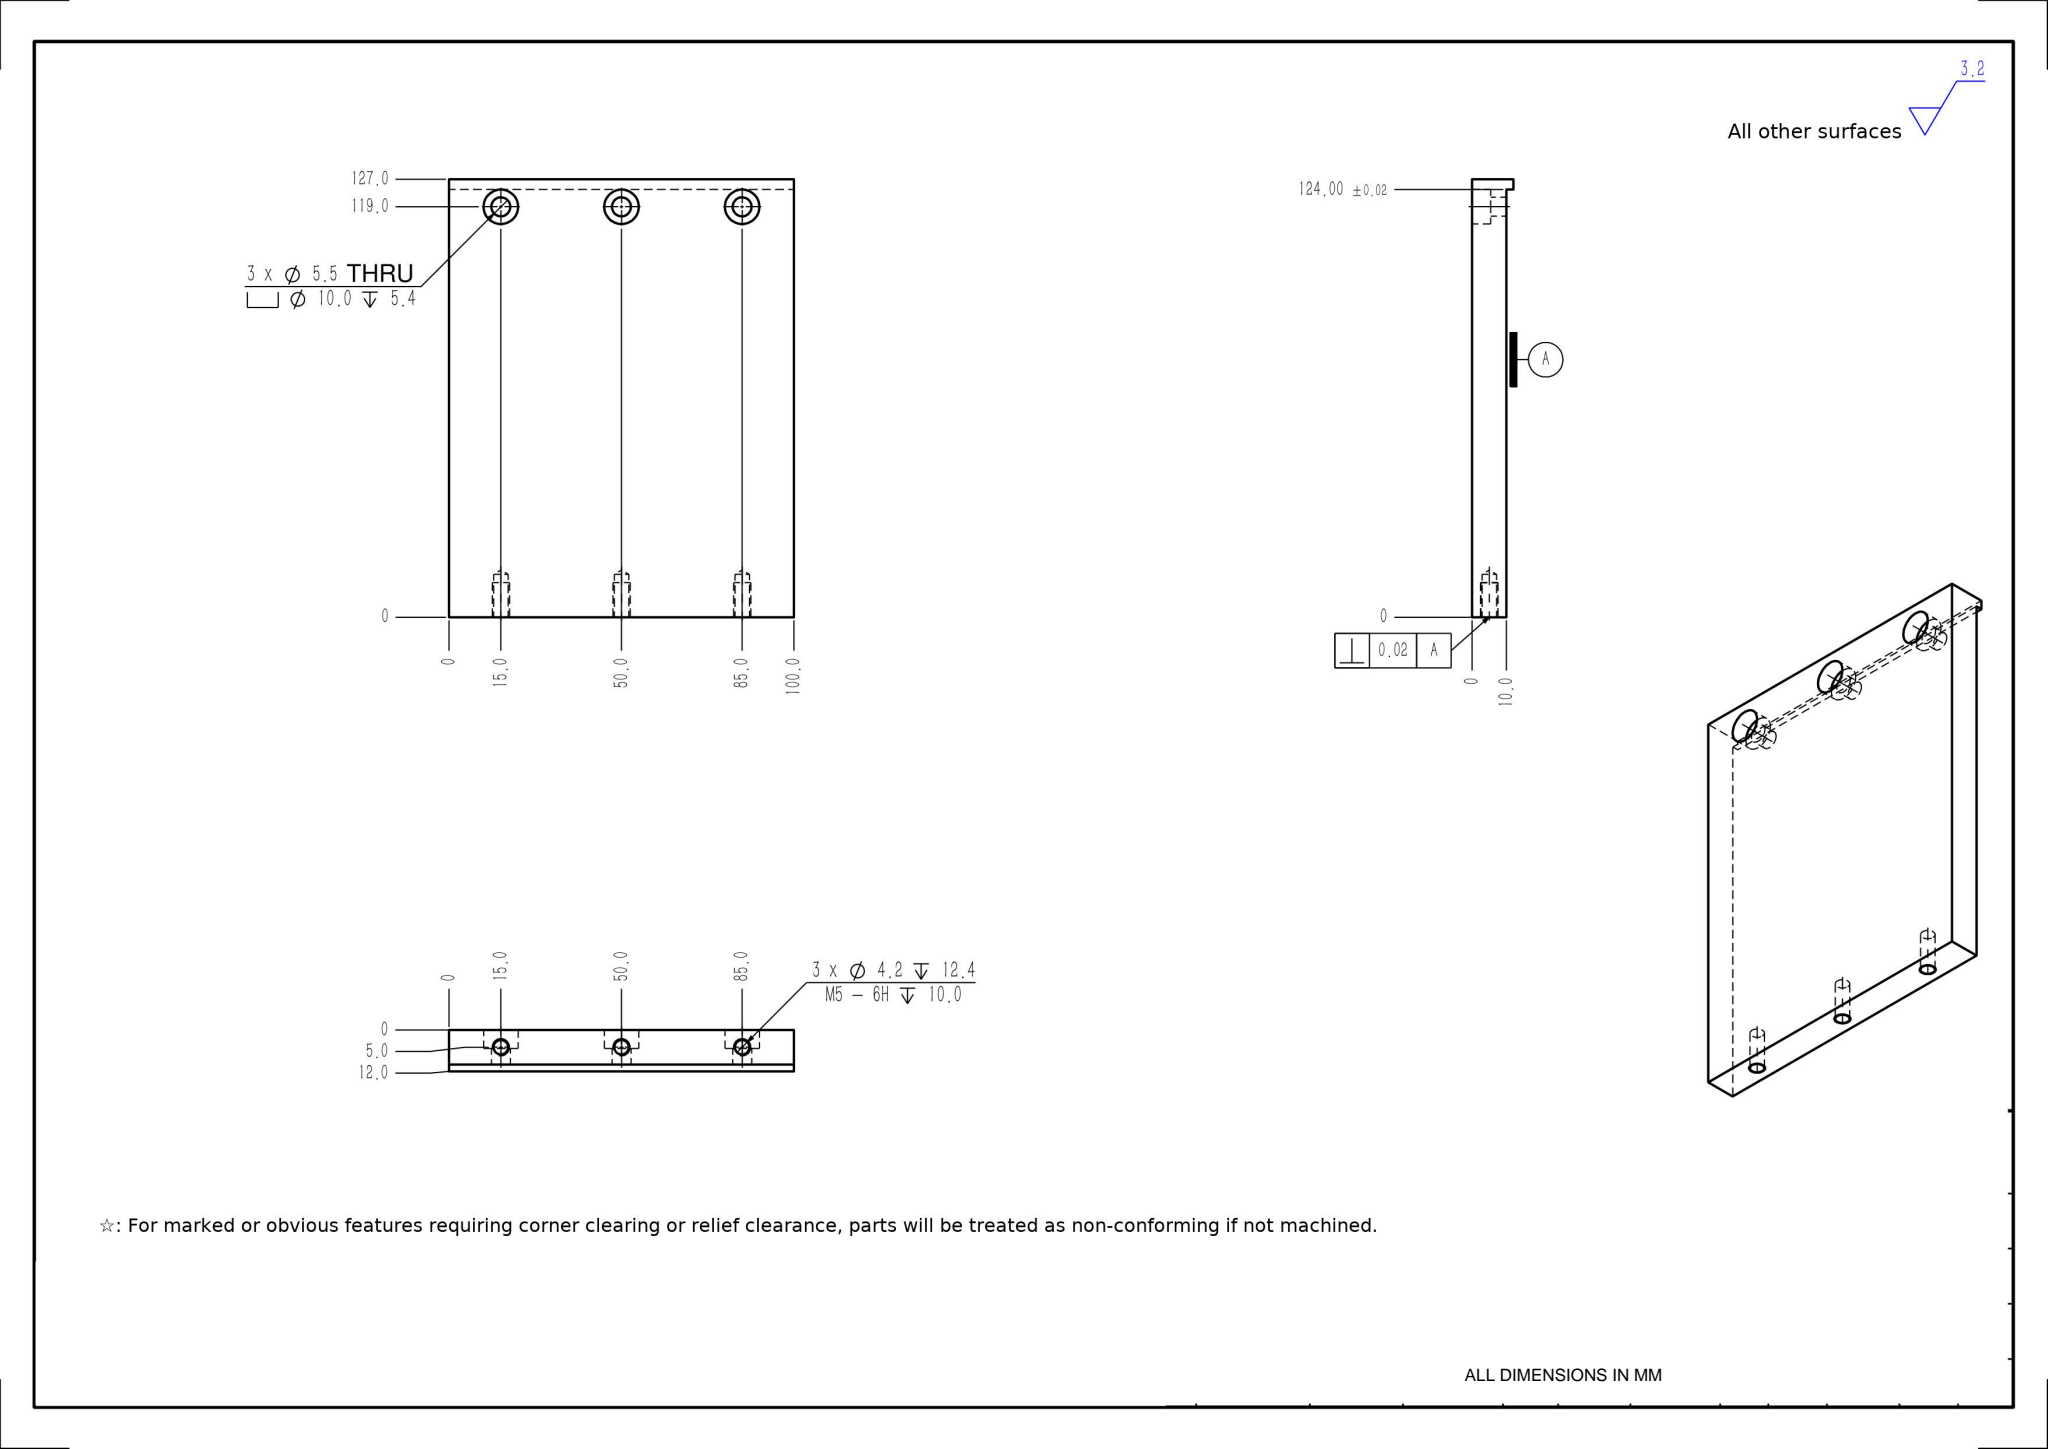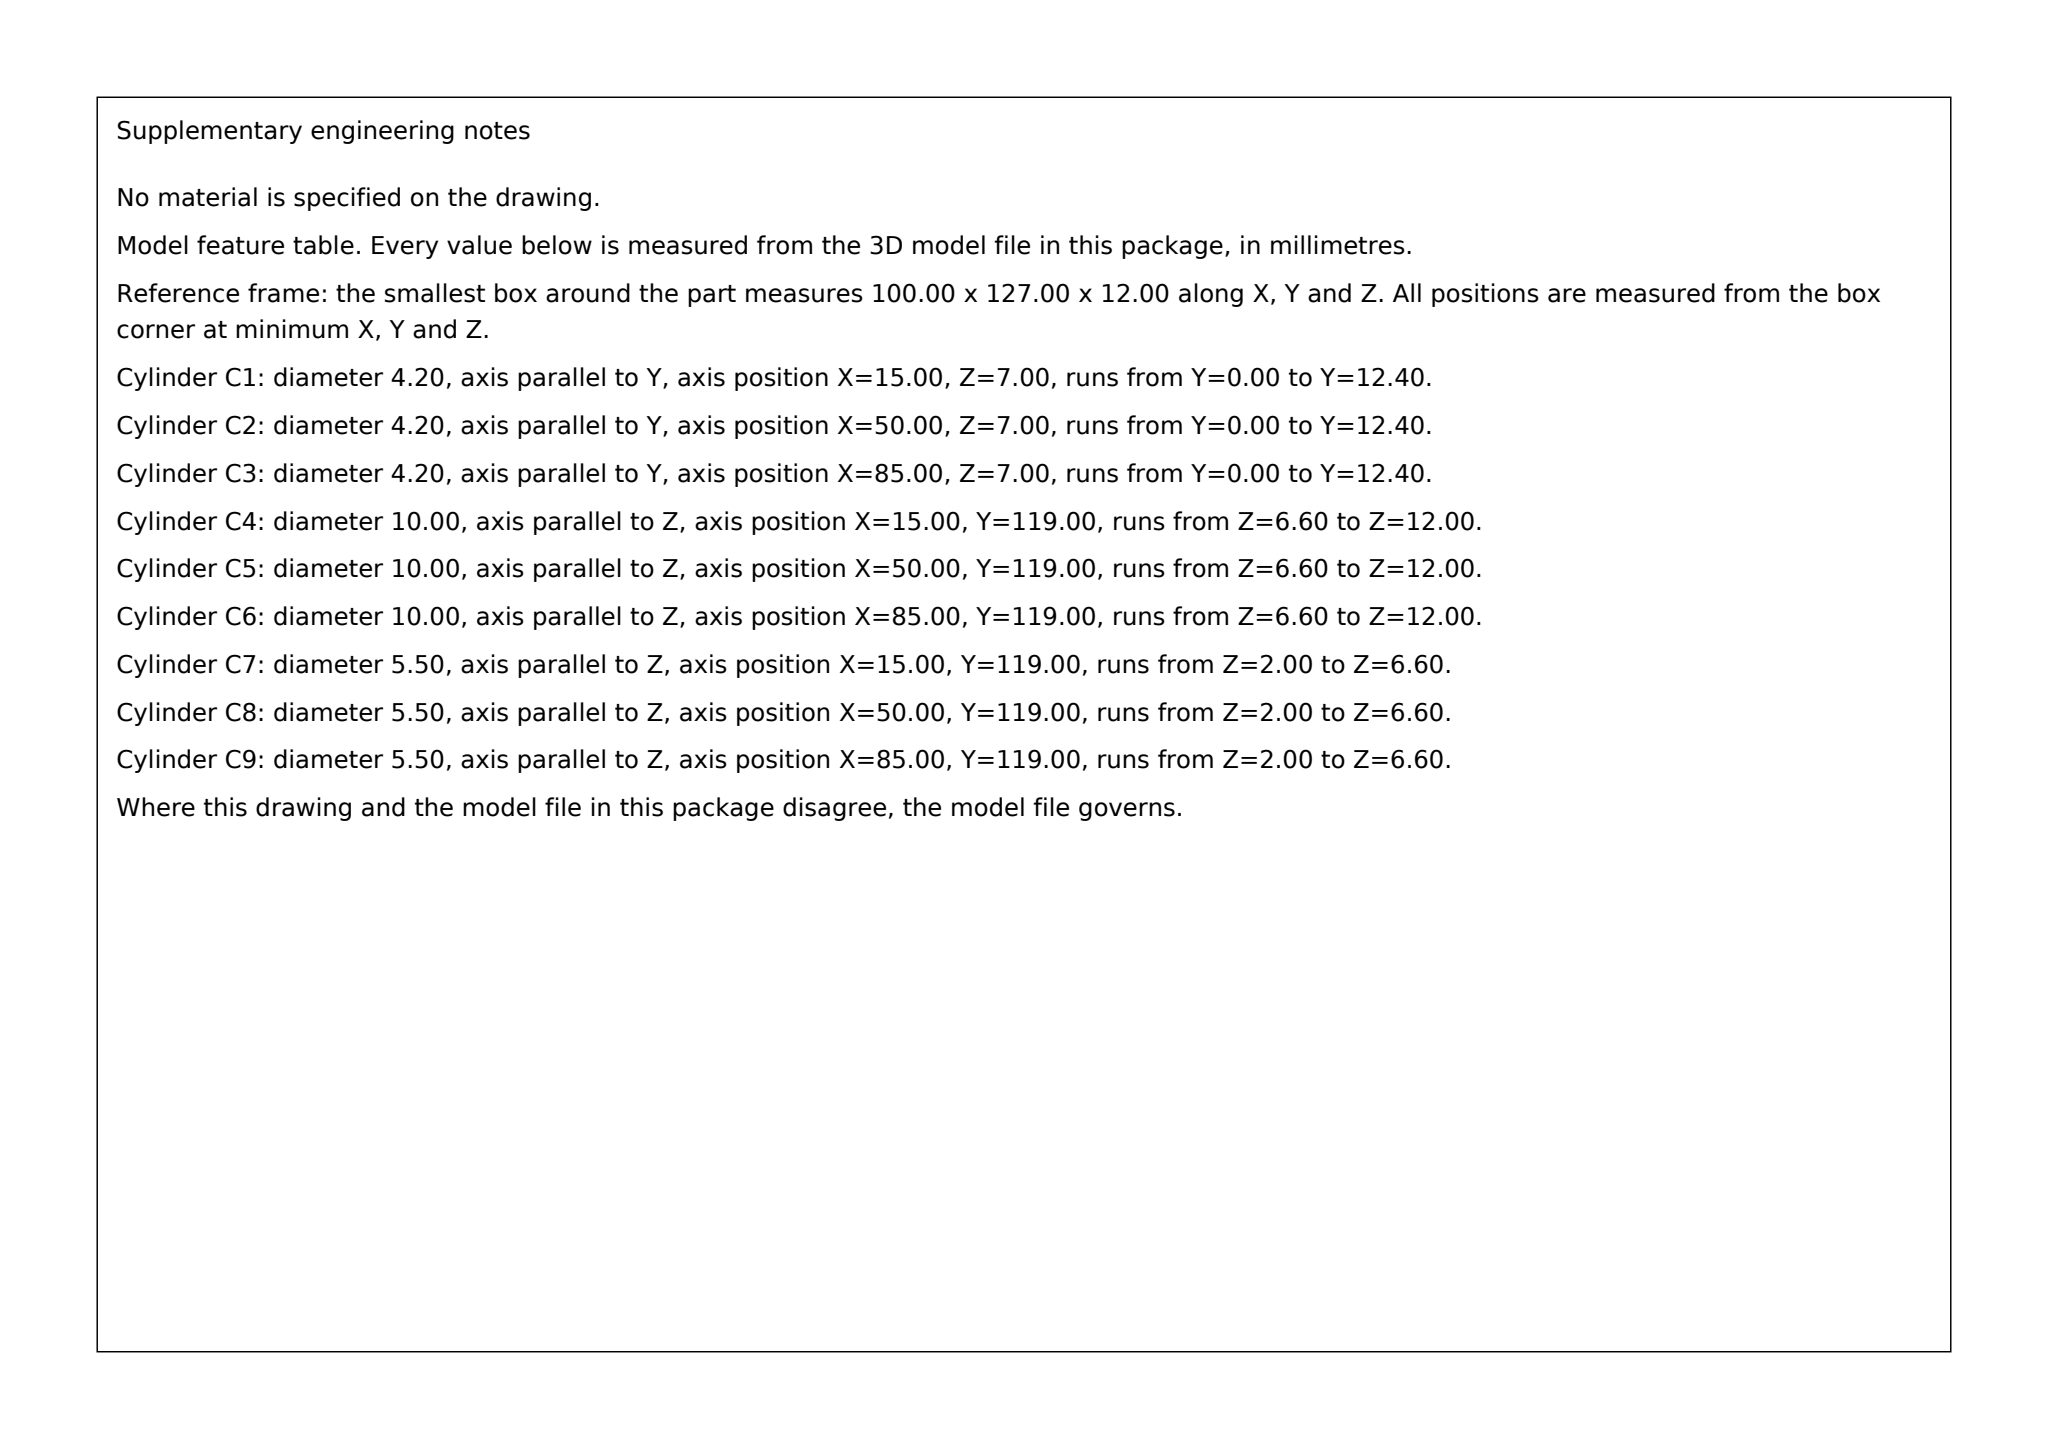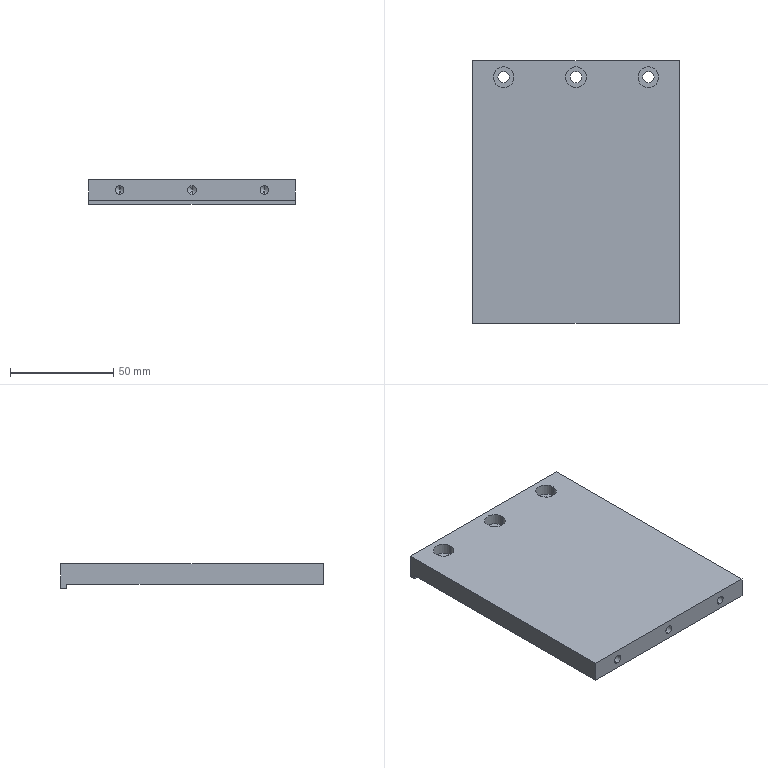Part | SolidWorks | mm | 1 solid | 35 faces | box 100 x 127 x 12 mm | volume 125467 mm3 | cylinder 18 | plane 11 | cone 6 | commonest cylinder face diameters 4.2 x6 10 x6 5.5 x6
build123d program:
from build123d import *

# Parameters (mm, degrees)
SKETCH1_W                                       = 100
SKETCH1_H                                       = 127
BOSS_EXTRUDE1_DEPTH                             = 6
SKETCH2_W                                       = 100
SKETCH2_H                                       = 124
CUT_EXTRUDE1_DEPTH                              = 2
M5_HEX_SOCKET_HEAD_CAP_SCREW_CBORE1_D           = 5.5
M5_HEX_SOCKET_HEAD_CAP_SCREW_CBORE1_CBORE_D     = 10
M5_HEX_SOCKET_HEAD_CAP_SCREW_CBORE1_CBORE_DEPTH = 5.4
M5_TAPPED_HOLE1_D                               = 4.2
M5_TAPPED_HOLE1_DEPTH                           = 12.4
M5_TAPPED_HOLE1_TIP                             = 1.262


with BuildPart() as part:
    # Sketch1 → Boss-Extrude1 (new, symmetric)
    with BuildSketch(Plane.XY):
        Rectangle(SKETCH1_W, SKETCH1_H)
    extrude(amount=BOSS_EXTRUDE1_DEPTH, both=True)

    # Sketch2 → Cut-Extrude1 (cut)
    with BuildSketch(Plane(origin=(0, 0, -6), x_dir=(-1, 0, 0), z_dir=(0, 0, -1))):
        with Locations((0, -1.5)):
            Rectangle(SKETCH2_W, SKETCH2_H)
    extrude(amount=-CUT_EXTRUDE1_DEPTH, mode=Mode.SUBTRACT)

    # M5 Hex Socket Head Cap Screw CBORE1 (through all)
    with Locations(Plane.XY.offset(6)):
        with Locations((35, 55.5), (0, 55.5), (-35, 55.5)):
            CounterBoreHole(M5_HEX_SOCKET_HEAD_CAP_SCREW_CBORE1_D / 2, M5_HEX_SOCKET_HEAD_CAP_SCREW_CBORE1_CBORE_D / 2, M5_HEX_SOCKET_HEAD_CAP_SCREW_CBORE1_CBORE_DEPTH)

    # M5 Tapped Hole1
    with Locations(Plane(origin=(0, -63.5, 0), x_dir=(-1, 0, 0), z_dir=(0, -1, 0))):
        with Locations((0, -1), (35, -1), (-35, -1)):
            Hole(M5_TAPPED_HOLE1_D / 2, depth=M5_TAPPED_HOLE1_DEPTH)
            with Locations((0, 0, -(M5_TAPPED_HOLE1_DEPTH + M5_TAPPED_HOLE1_TIP / 2))):  # 118° drill point
                Cone(0, M5_TAPPED_HOLE1_D / 2, M5_TAPPED_HOLE1_TIP, mode=Mode.SUBTRACT)


solid = part.part